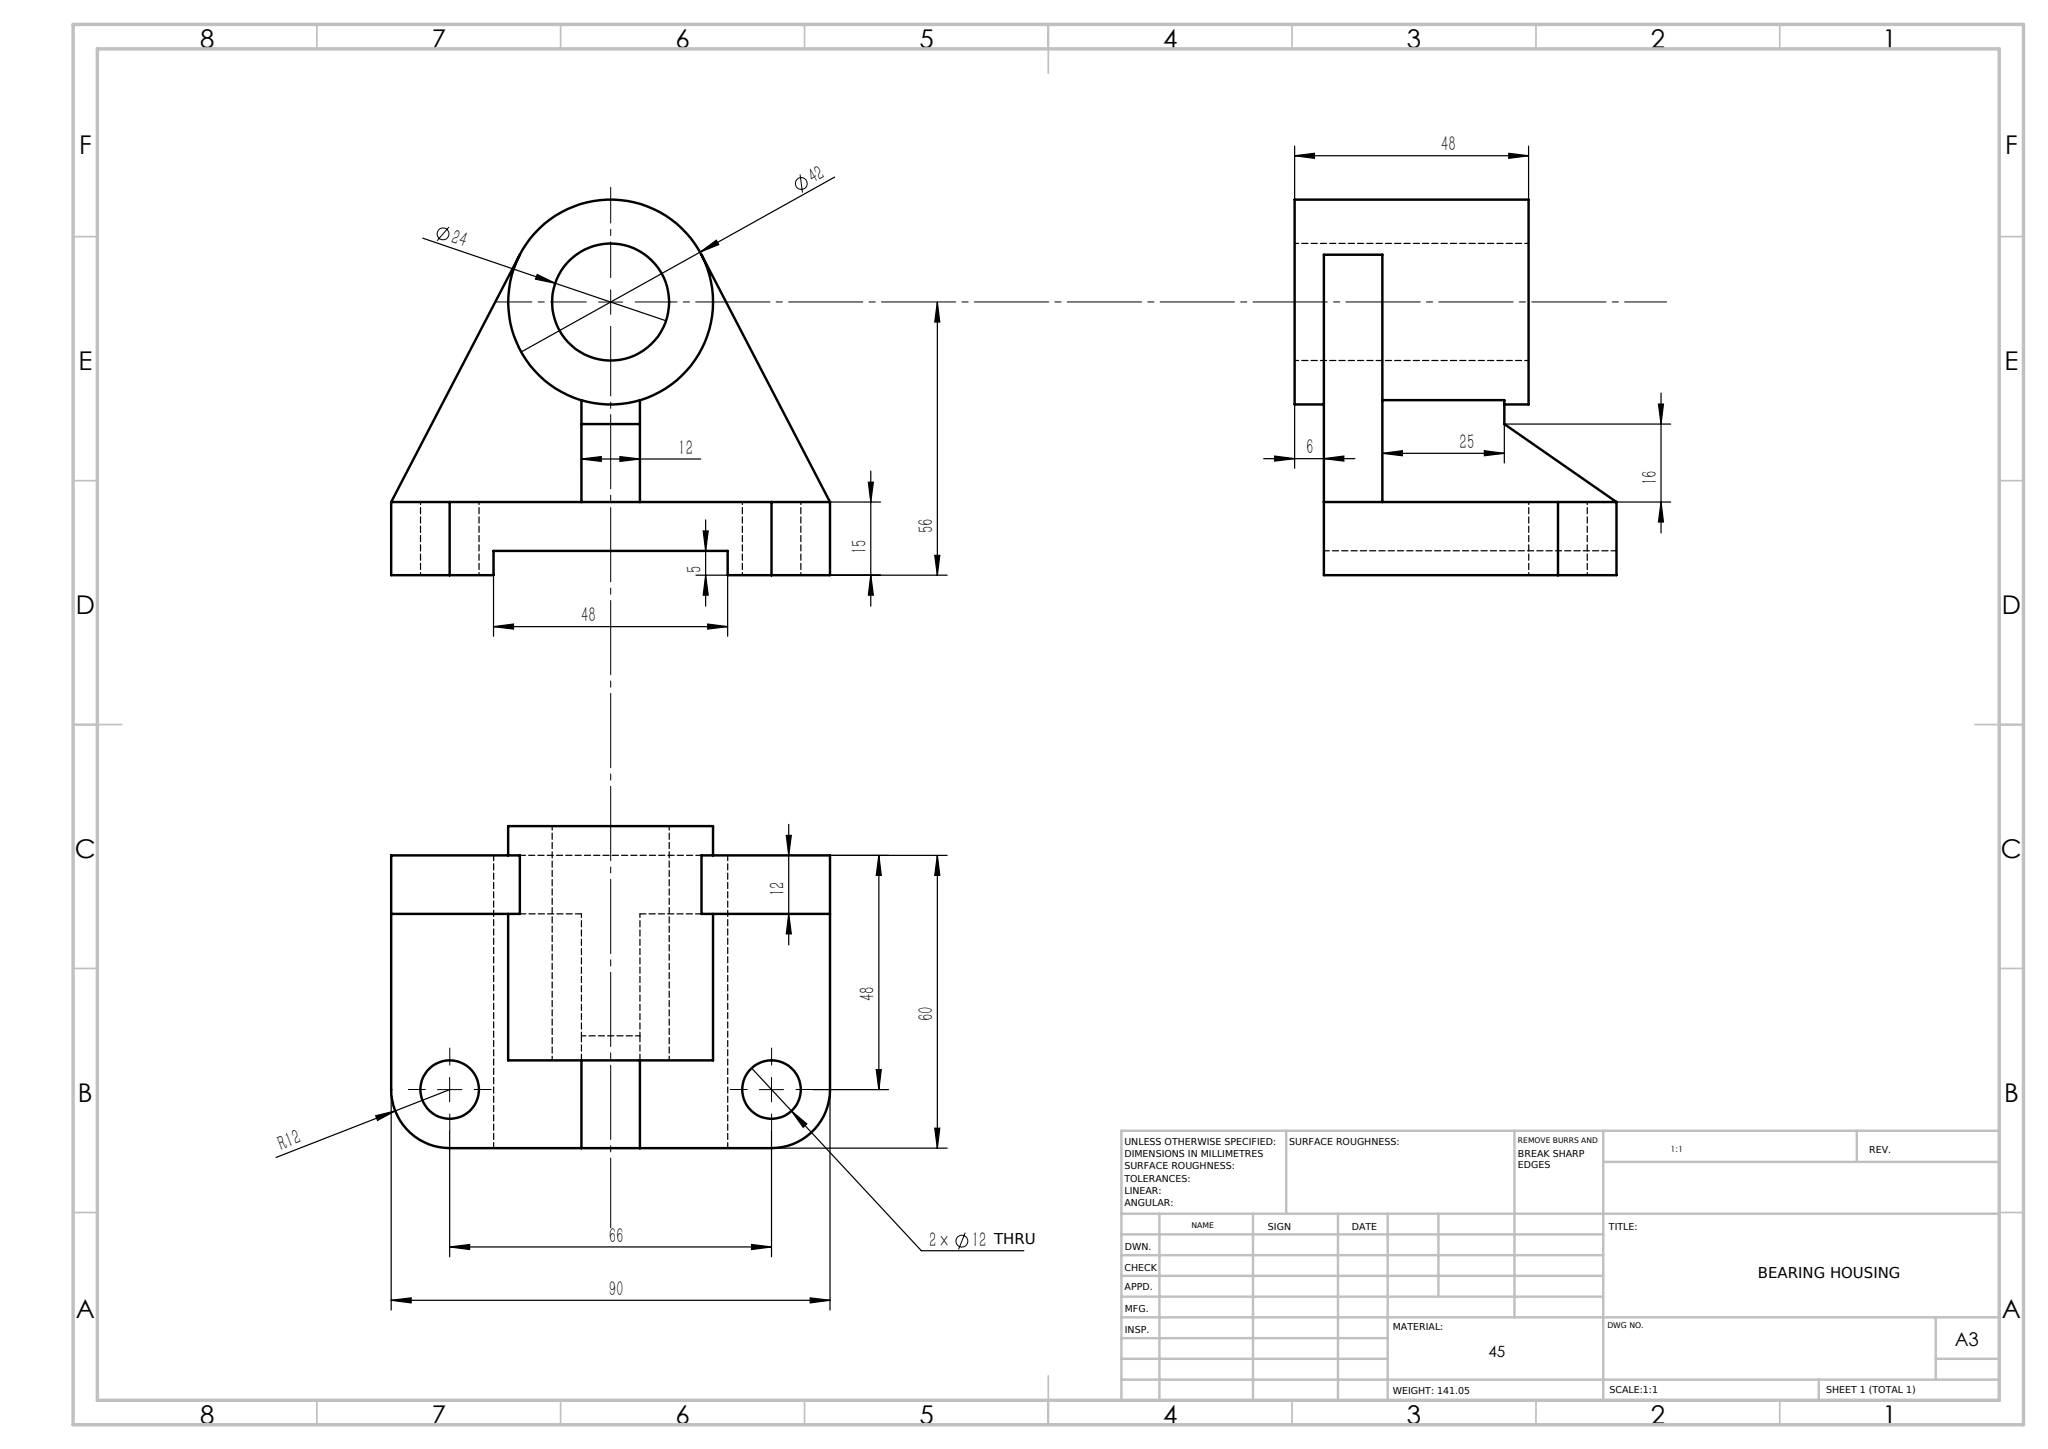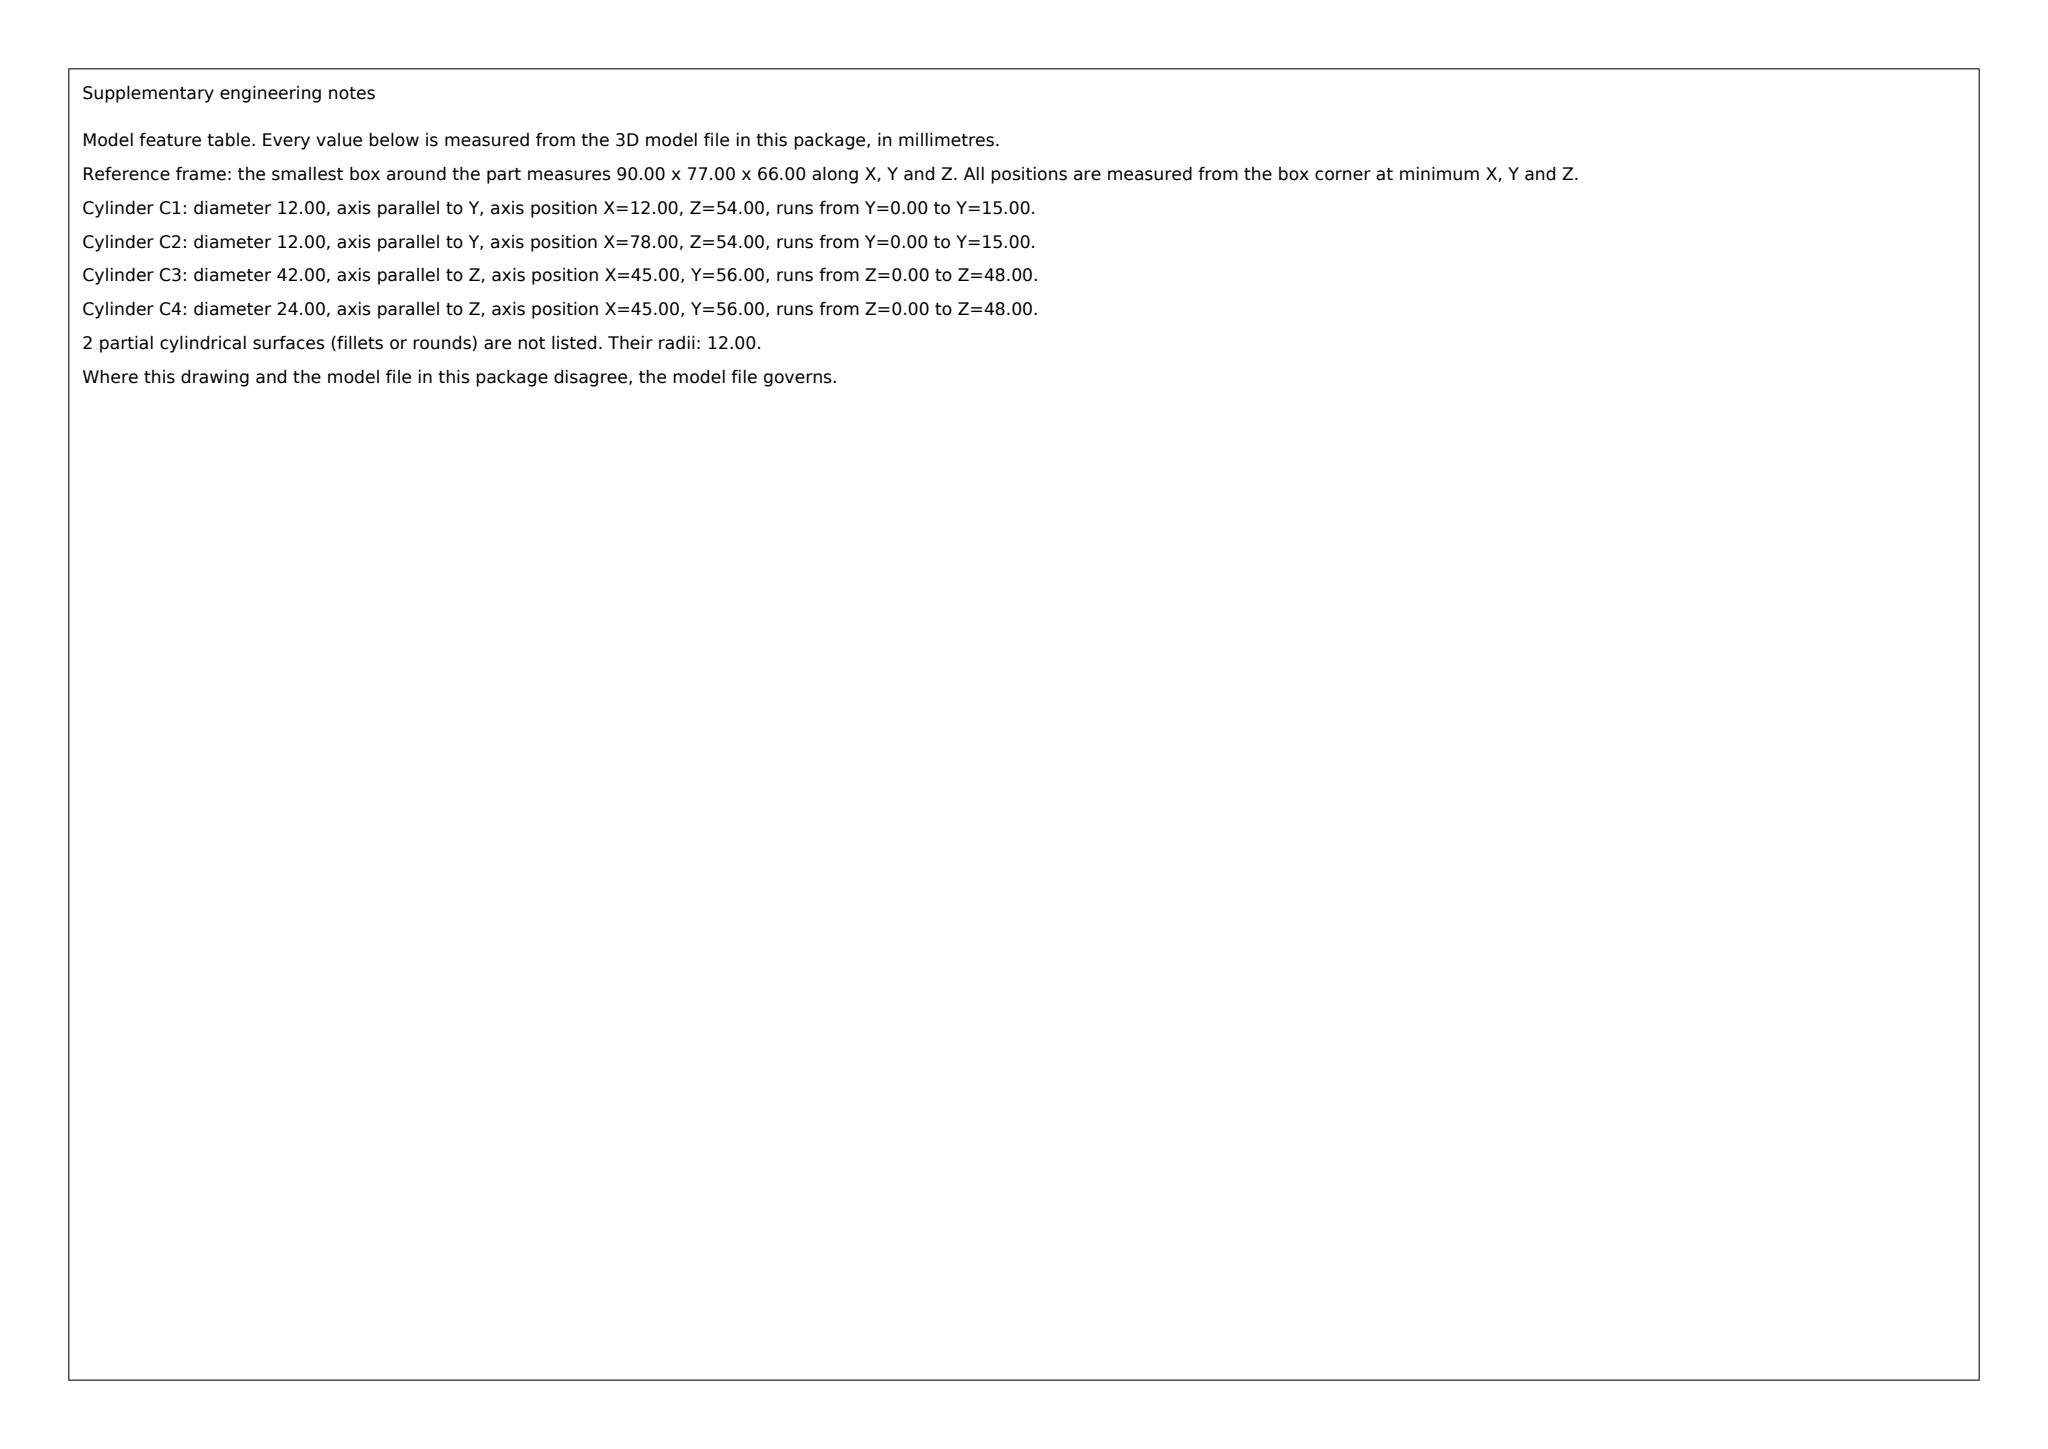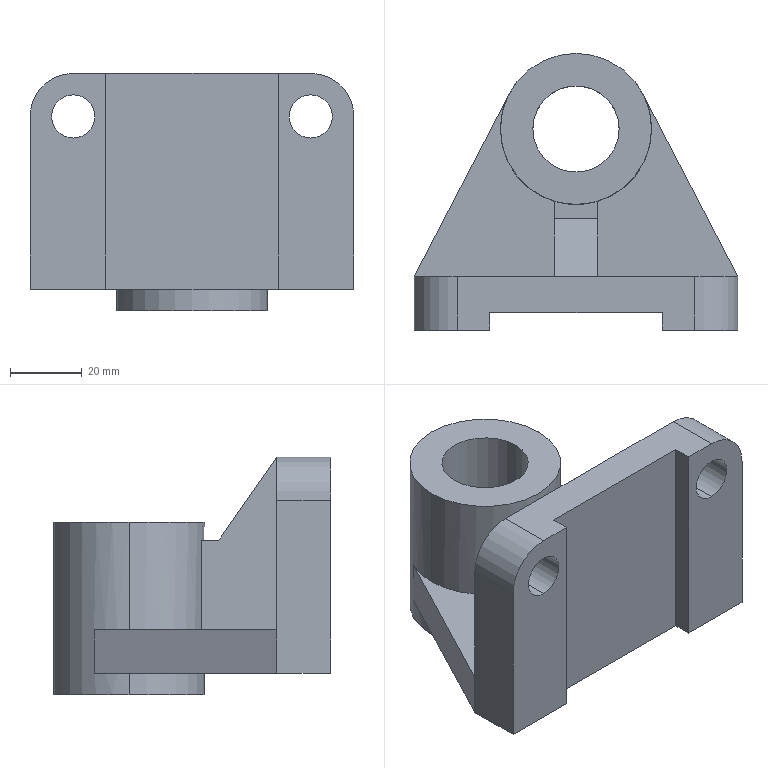Part | SolidWorks | mm | 1 solid | 32 faces | box 90 x 77 x 66 mm | volume 141050 mm3 | plane 21 | cylinder 11 | commonest cylinder face diameters 24 x4 12 x4 42 x3